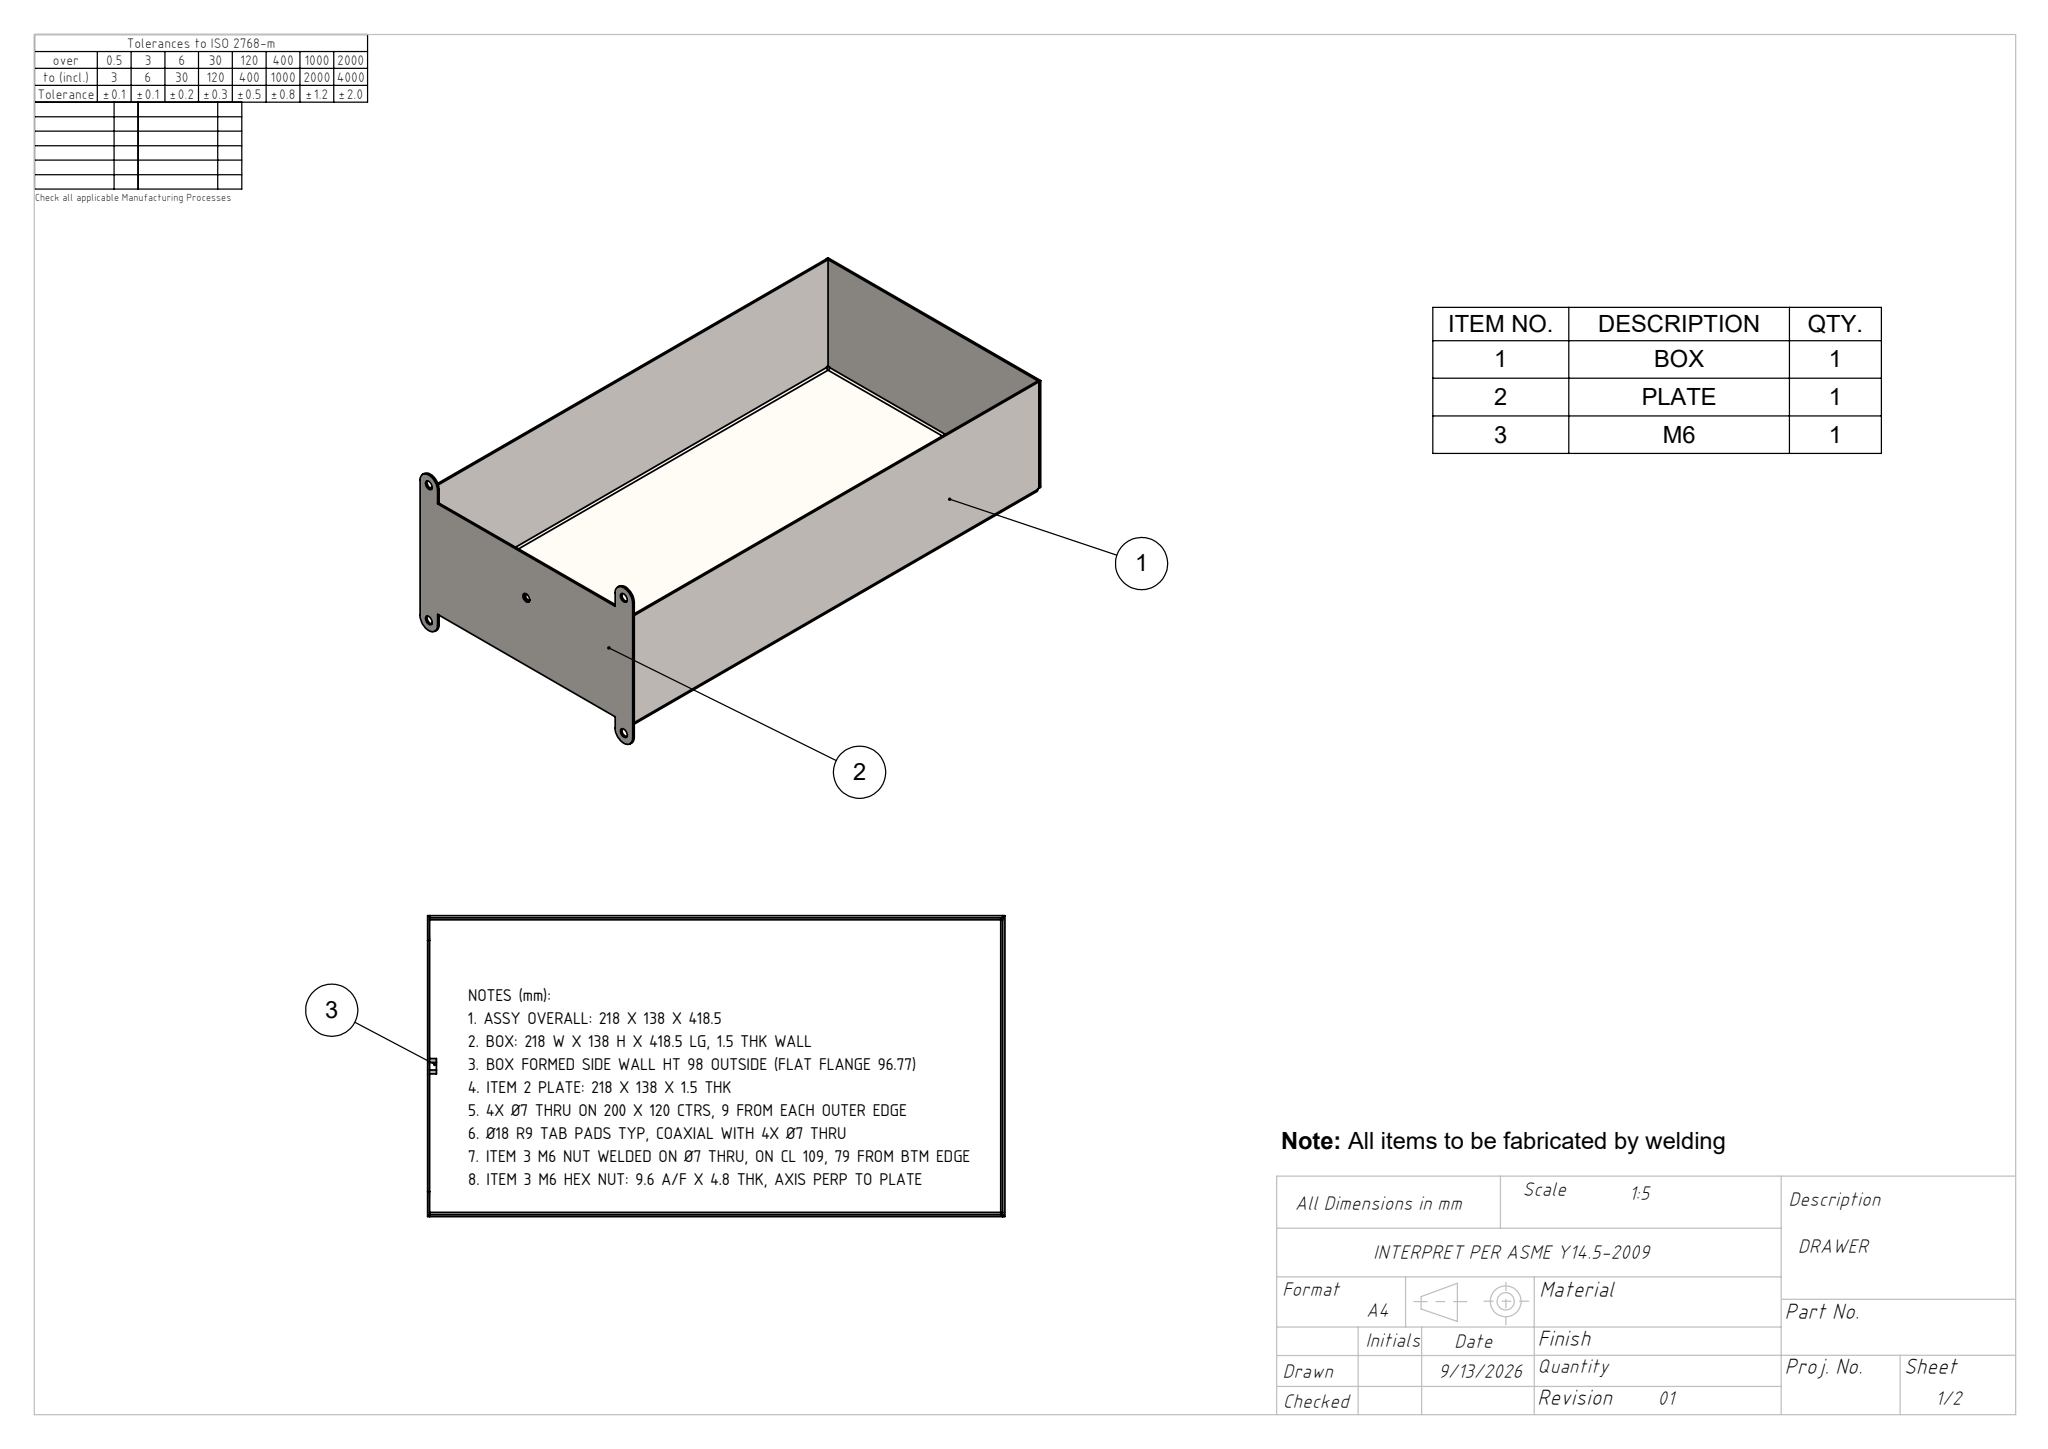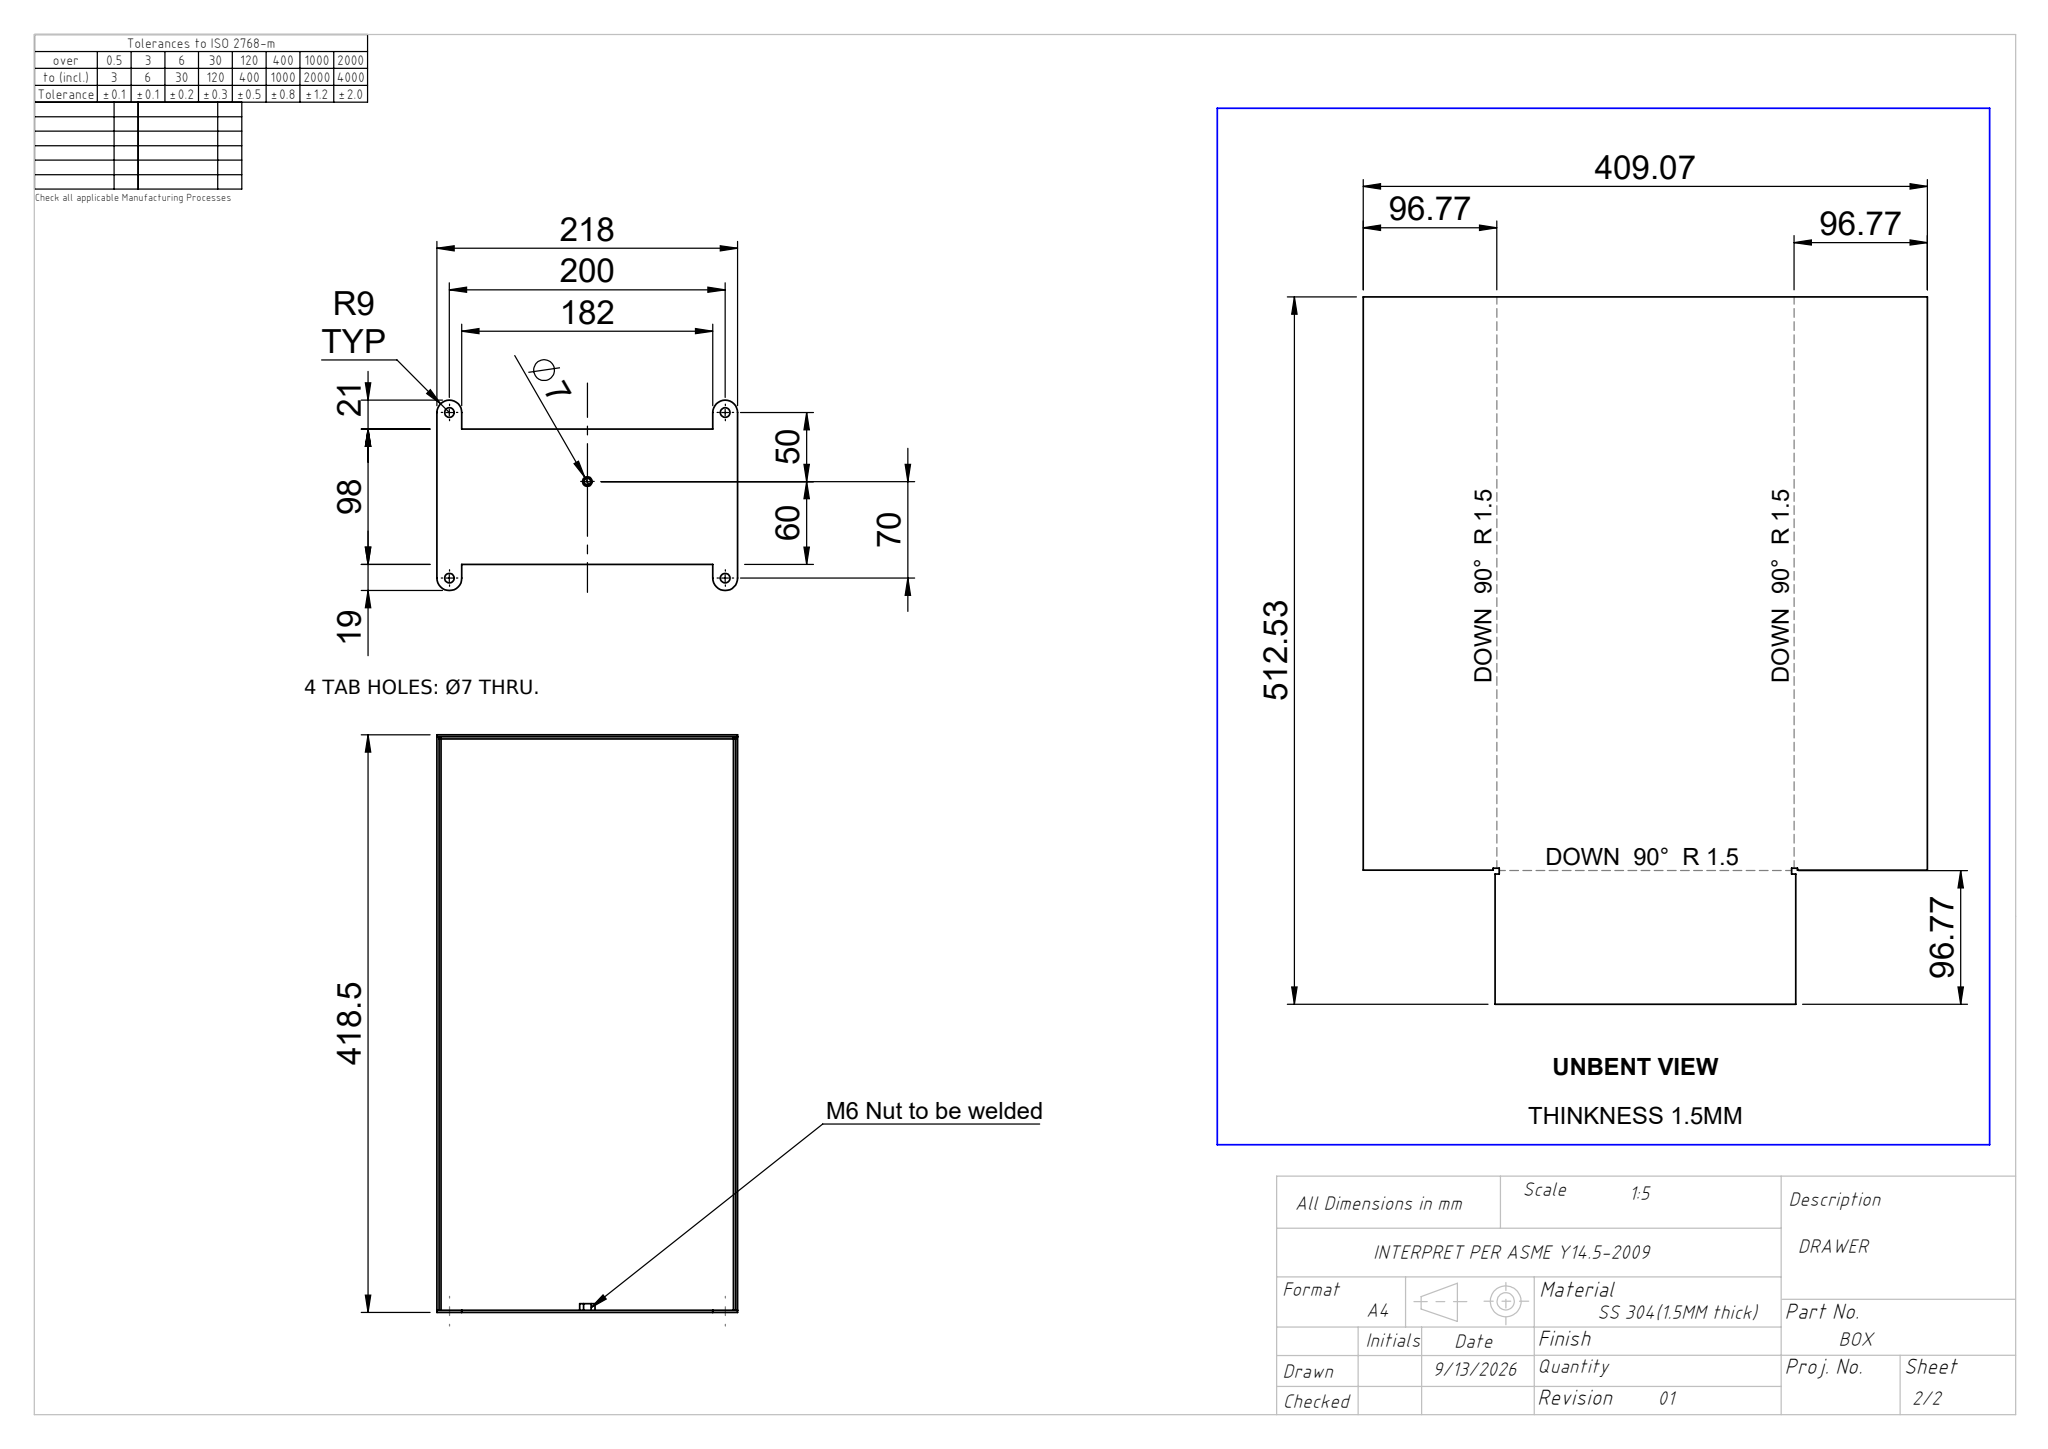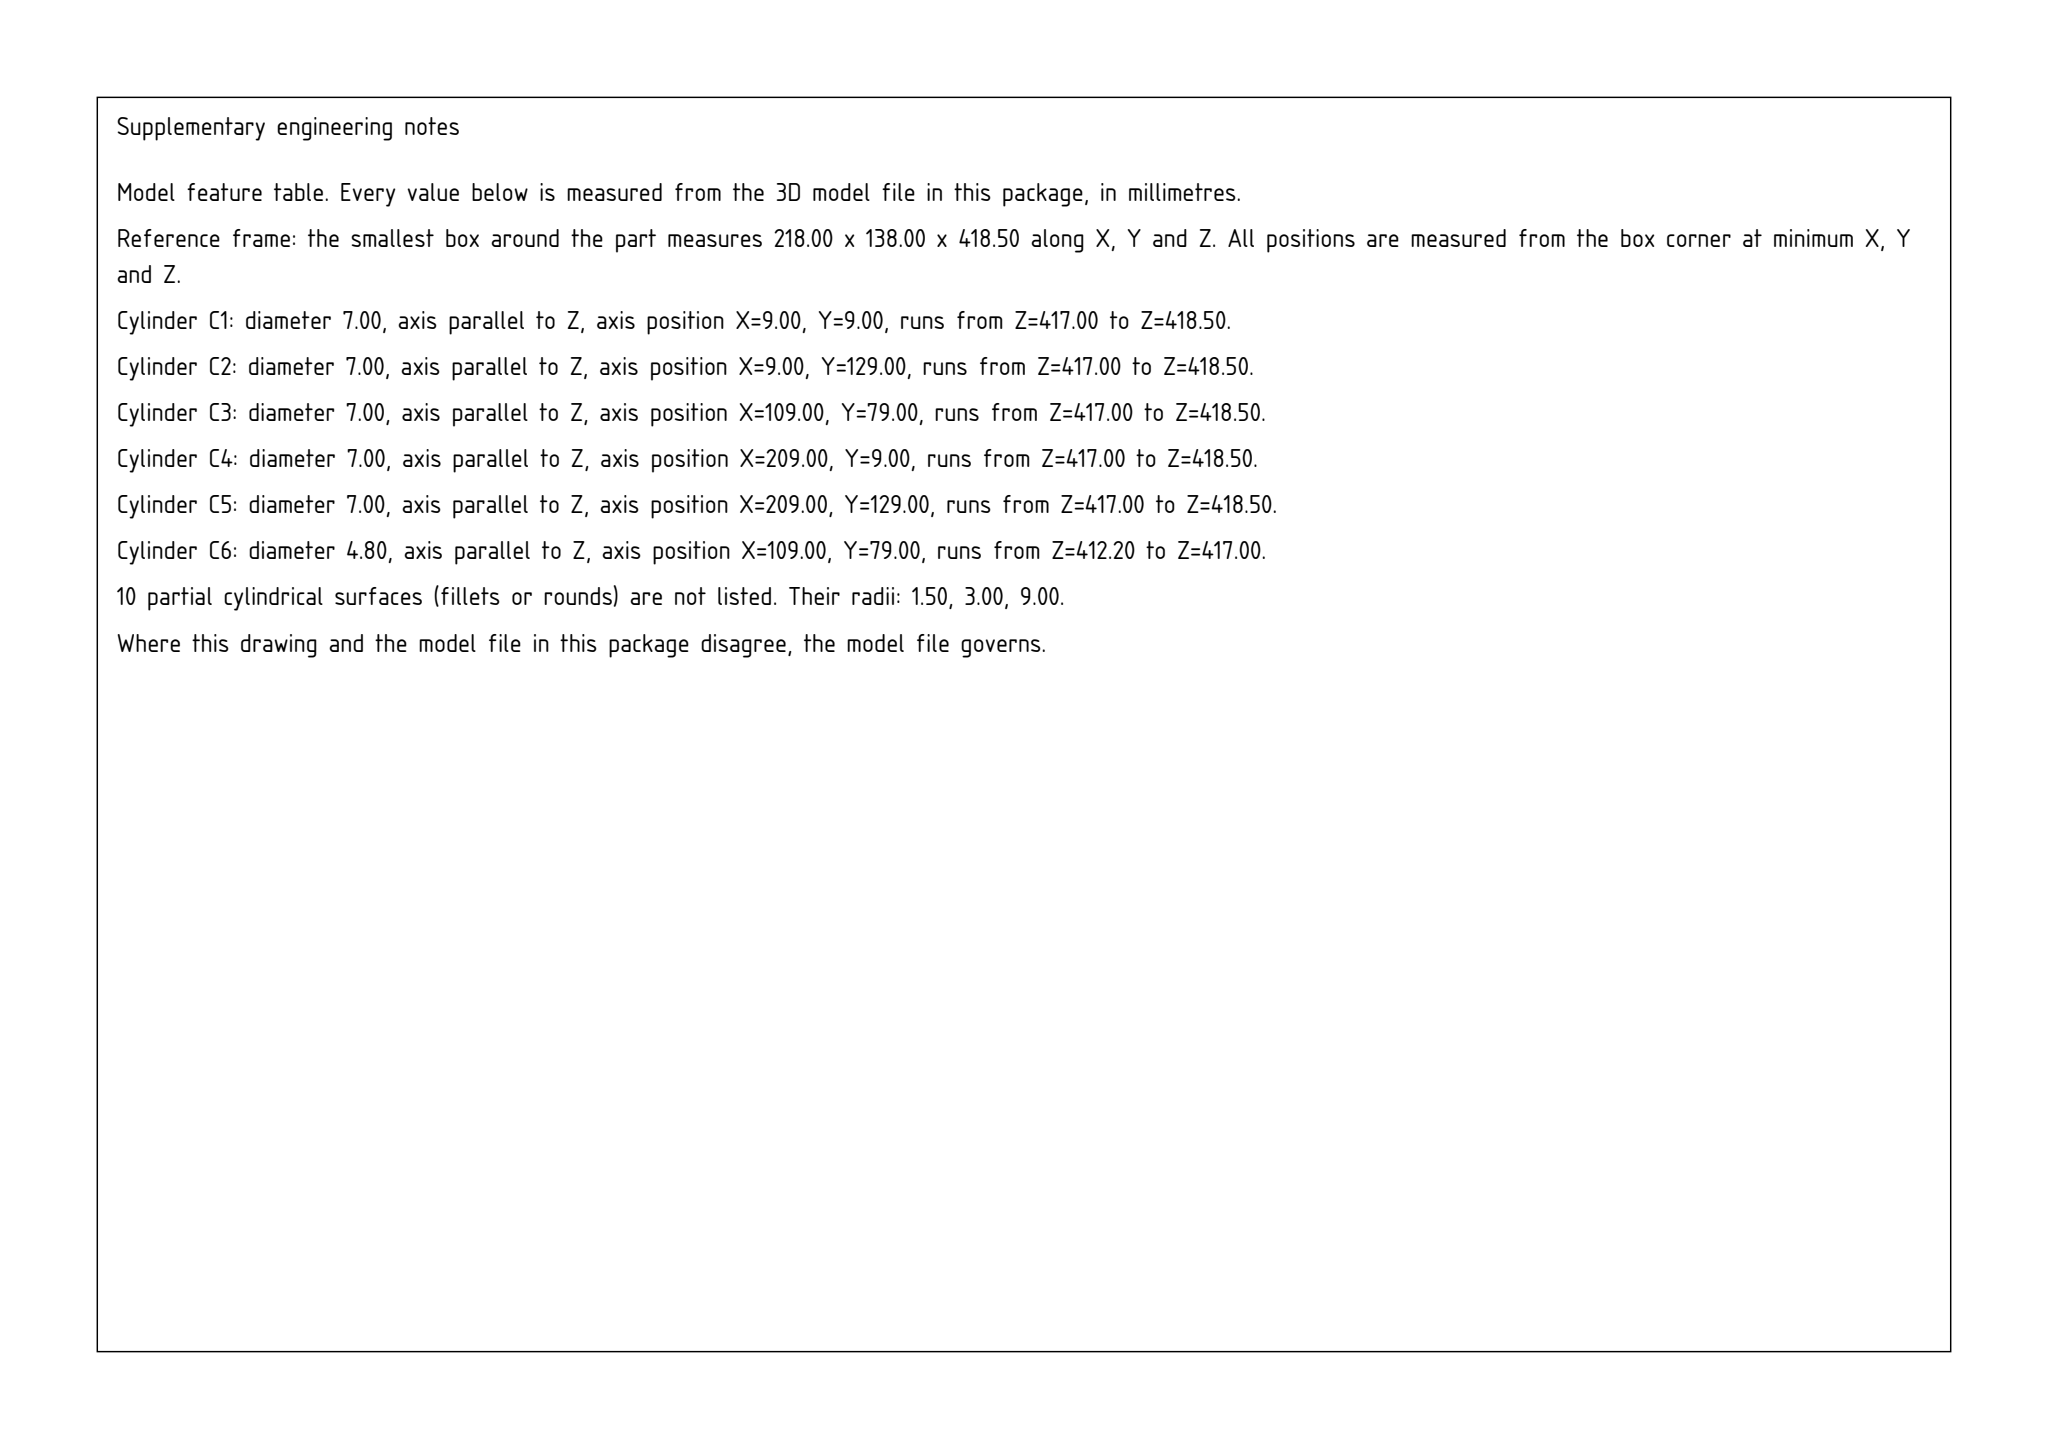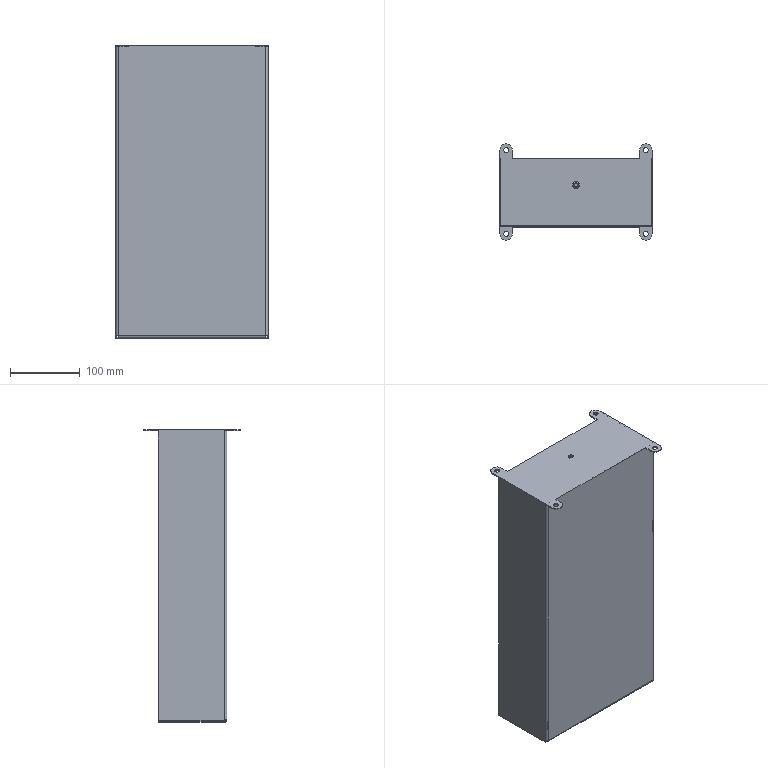Part | SolidWorks | mm | 1 solid | 66 faces | box 218 x 138 x 418.5 mm | volume 320614 mm3 | plane 44 | cylinder 22 | commonest cylinder face diameters 7 x10 18 x4 6 x3 3 x3 4.8 x2
Drawing notes:
ASSY OVERALL: 218 X 138 X 418.5 | from the solid: bbox_xyz 218.0, 138.0, 418.5
BOX: 218 W X 138 H X 418.5 LG, 1.5 THK WALL | from the solid: bbox 218x138x418.5; x planes 0/1.5 and 216.5/218 = 1.5 wall
BOX FORMED SIDE WALL HT 98 OUTSIDE (FLAT FLANGE 96.77) | from the solid: Y planes 19.0 and 117.0 bound box walls: 117-19 = 98 formed ht
ITEM 2 PLATE: 218 X 138 X 1.5 THK | from the solid: plate bbox X0-218, Y0-138, 1.5 thk (z planes 0/1.5)
4X Ø7 THRU ON 200 X 120 CTRS, 9 FROM EACH OUTER EDGE | from the solid: Ø7 z-holes len 1.5 at (9,9)(209,9)(9,129)(209,129) = 200 x 120 ctrs
Ø18 R9 TAB PADS TYP, COAXIAL WITH 4X Ø7 THRU | from the solid: Ø18 z-features len 1.5 at same 4 hole ctrs = R9 tabs
ITEM 3 M6 NUT WELDED ON Ø7 THRU, ON CL 109, 79 FROM BTM EDGE | from the solid: Ø7 z-hole at (109,79) = CL of 218; Ø4.8 nut bore coaxial
ITEM 3 M6 HEX NUT: 9.6 A/F X 4.8 THK, AXIS PERP TO PLATE | from the solid: Y planes 74.2 & 83.8 = 9.6 A/F about nut ctr Y79; Ø4.8 z-cyl len 4.8